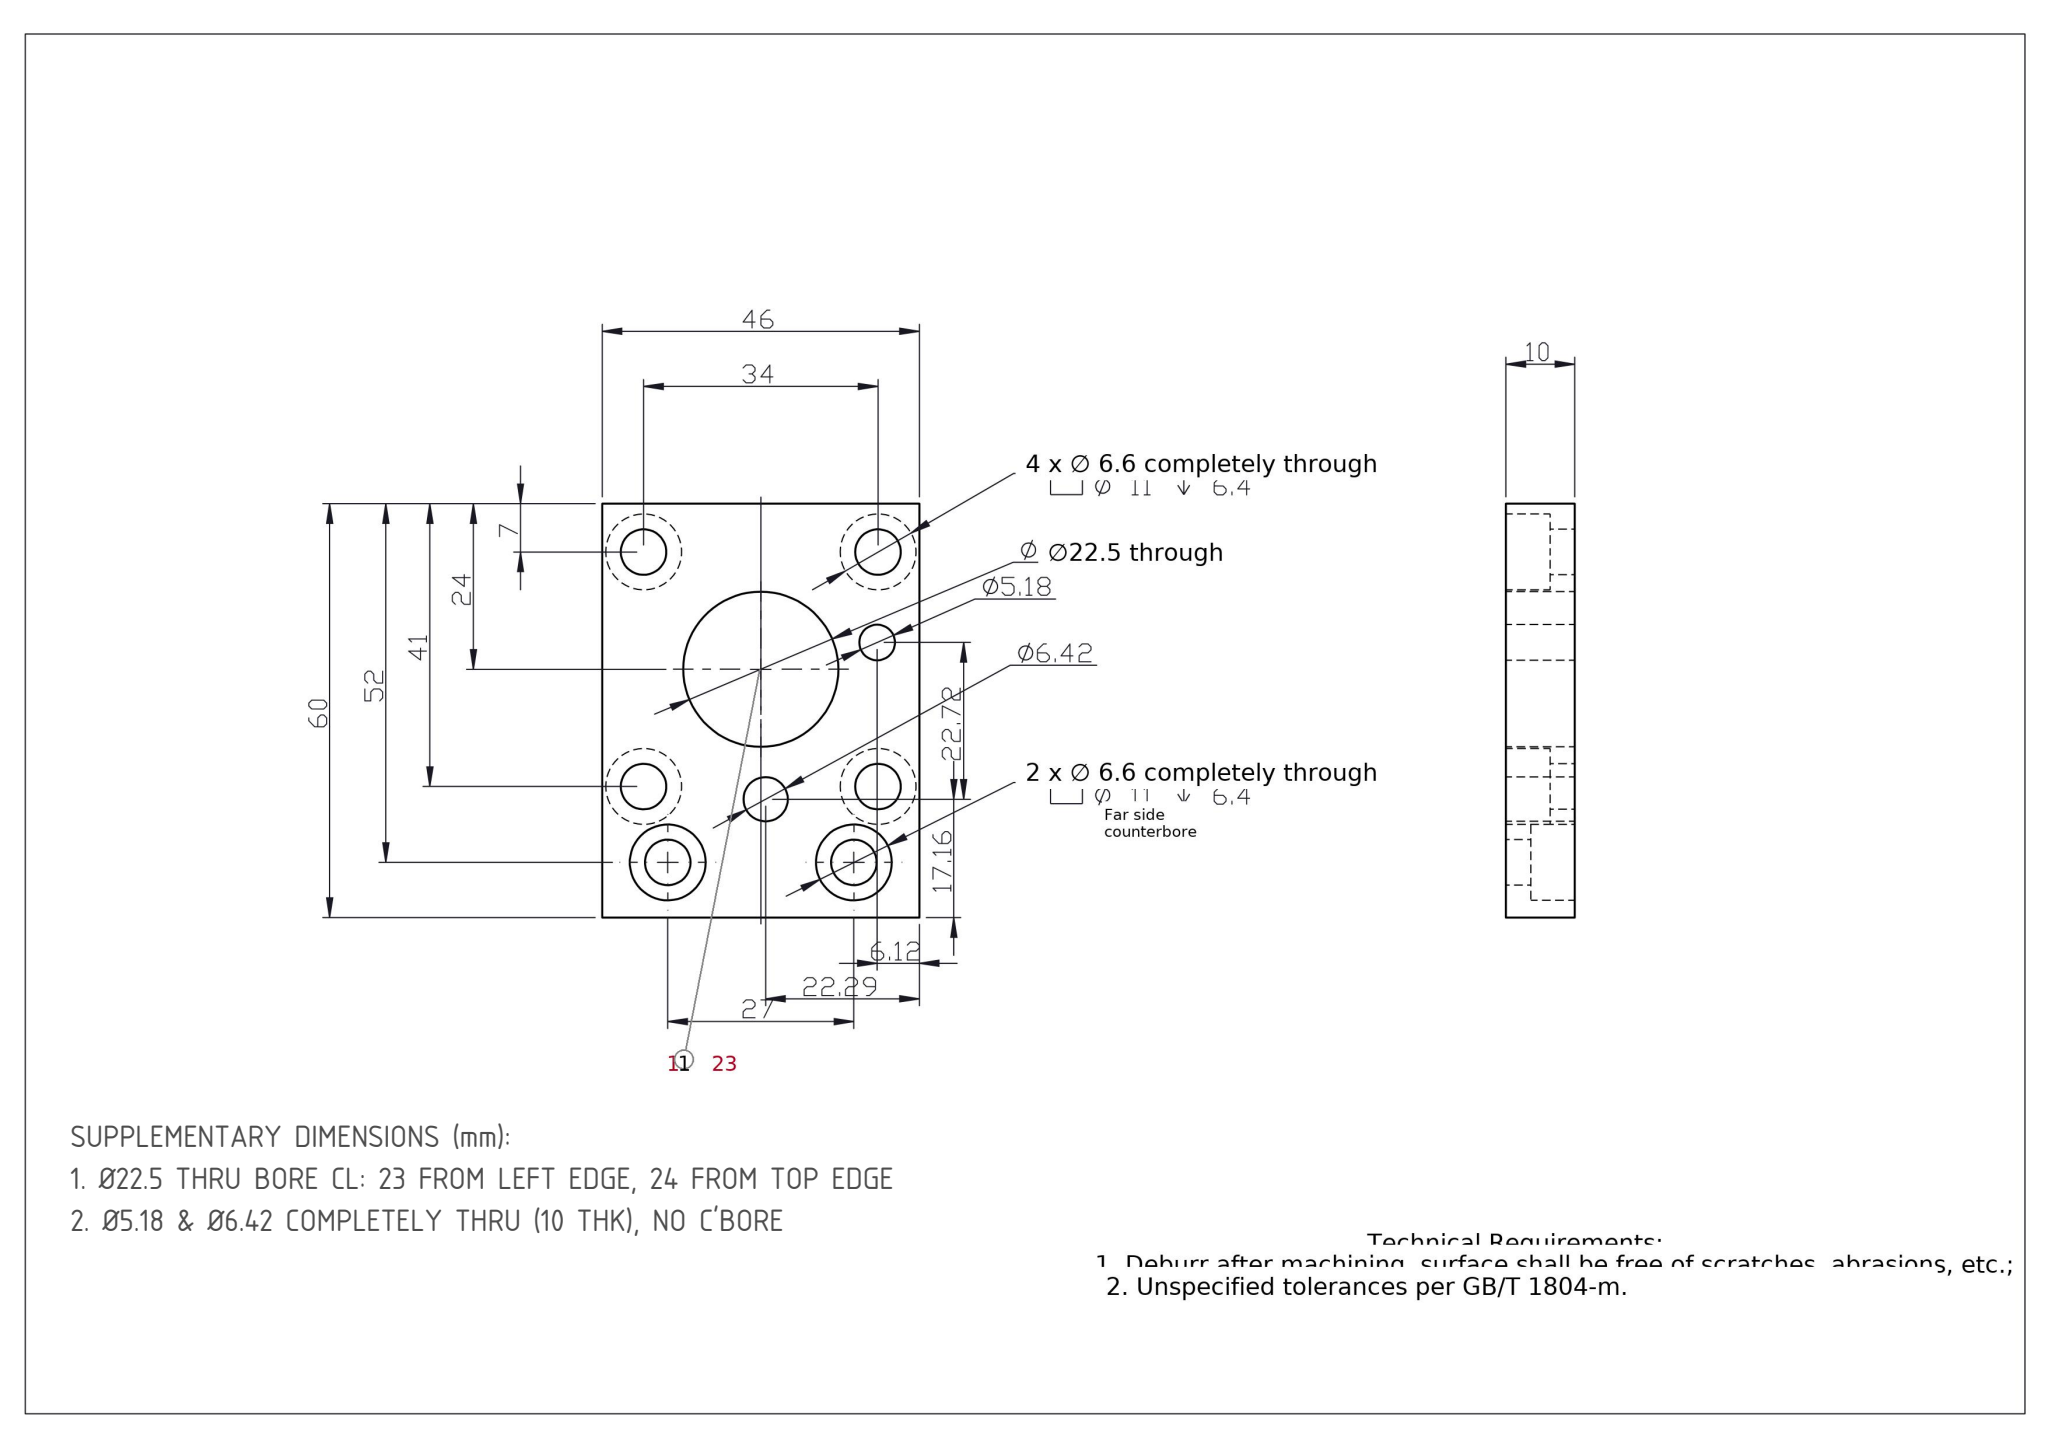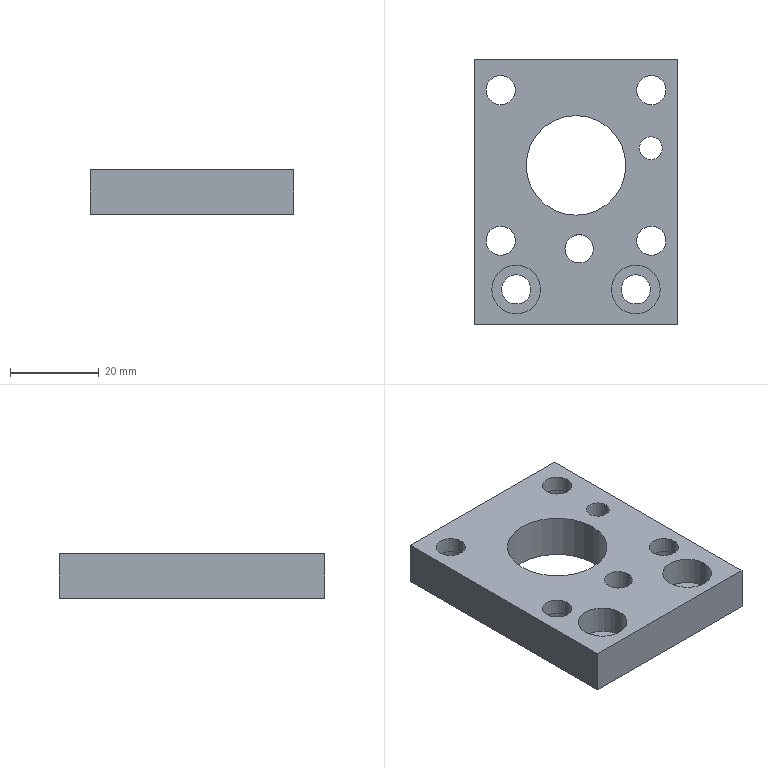Part | SolidWorks | mm | 1 solid | 42 faces | box 46 x 60 x 10 mm | volume 18701 mm3 | cylinder 30 | plane 12 | commonest cylinder face diameters 11 x12 6.6 x12 5.177 x2 6.422 x2 22.5 x2
build123d program:
from build123d import *

# Parameters (mm, degrees)
SKETCH1_W                                       = 46
SKETCH1_H                                       = 60
BOSS_EXTRUDE1_DEPTH                             = 10
M6_HEX_SOCKET_HEAD_CAP_SCREW_CBORE1_D           = 6.6
M6_HEX_SOCKET_HEAD_CAP_SCREW_CBORE1_CBORE_D     = 11
M6_HEX_SOCKET_HEAD_CAP_SCREW_CBORE1_CBORE_DEPTH = 6.4
M6_HEX_SOCKET_HEAD_CAP_SCREW_CBORE4_D           = 6.6
M6_HEX_SOCKET_HEAD_CAP_SCREW_CBORE4_CBORE_D     = 11
M6_HEX_SOCKET_HEAD_CAP_SCREW_CBORE4_CBORE_DEPTH = 6.4
SKETCH6_R                                       = 11.25
CUT_EXTRUDE1_DEPTH                              = 77.263
SKETCH7_R                                       = 2.589
SKETCH7_R_2                                     = 3.211
CUT_EXTRUDE2_DEPTH                              = 10


with BuildPart() as part:
    # Sketch1 → Boss-Extrude1 (new body)
    with BuildSketch(Plane.XY):
        with Locations((23, -30)):
            Rectangle(SKETCH1_W, SKETCH1_H)
    extrude(amount=BOSS_EXTRUDE1_DEPTH)

    # M6 Hex Socket Head Cap Screw CBORE1 (through all)
    with Locations(Plane.XY.offset(10)):
        with Locations((9.5, -52), (36.5, -52)):
            CounterBoreHole(M6_HEX_SOCKET_HEAD_CAP_SCREW_CBORE1_D / 2, M6_HEX_SOCKET_HEAD_CAP_SCREW_CBORE1_CBORE_D / 2, M6_HEX_SOCKET_HEAD_CAP_SCREW_CBORE1_CBORE_DEPTH)

    # M6 Hex Socket Head Cap Screw CBORE4 (through all)
    with Locations(Plane(origin=(0, 0, 0), x_dir=(-1, 0, 0), z_dir=(0, 0, -1))):
        with Locations((-40, -7), (-6, -7), (-6, -41), (-40, -41)):
            CounterBoreHole(M6_HEX_SOCKET_HEAD_CAP_SCREW_CBORE4_D / 2, M6_HEX_SOCKET_HEAD_CAP_SCREW_CBORE4_CBORE_D / 2, M6_HEX_SOCKET_HEAD_CAP_SCREW_CBORE4_CBORE_DEPTH)

    # Sketch6 → Cut-Extrude1 (cut, through all)
    with BuildSketch(Plane.XY.offset(10)):
        with Locations((23, -24)):
            Circle(SKETCH6_R)
    extrude(amount=-CUT_EXTRUDE1_DEPTH, mode=Mode.SUBTRACT)

    # Sketch7 → Cut-Extrude2 (cut)
    with BuildSketch(Plane(origin=(0, 0, 0), x_dir=(-1, 0, 0), z_dir=(0, 0, -1))):
        with Locations((-39.878, -20.115)):
            Circle(SKETCH7_R)
        with Locations((-23.708, -42.836)):
            Circle(SKETCH7_R_2)
    extrude(amount=-CUT_EXTRUDE2_DEPTH, mode=Mode.SUBTRACT)


solid = part.part